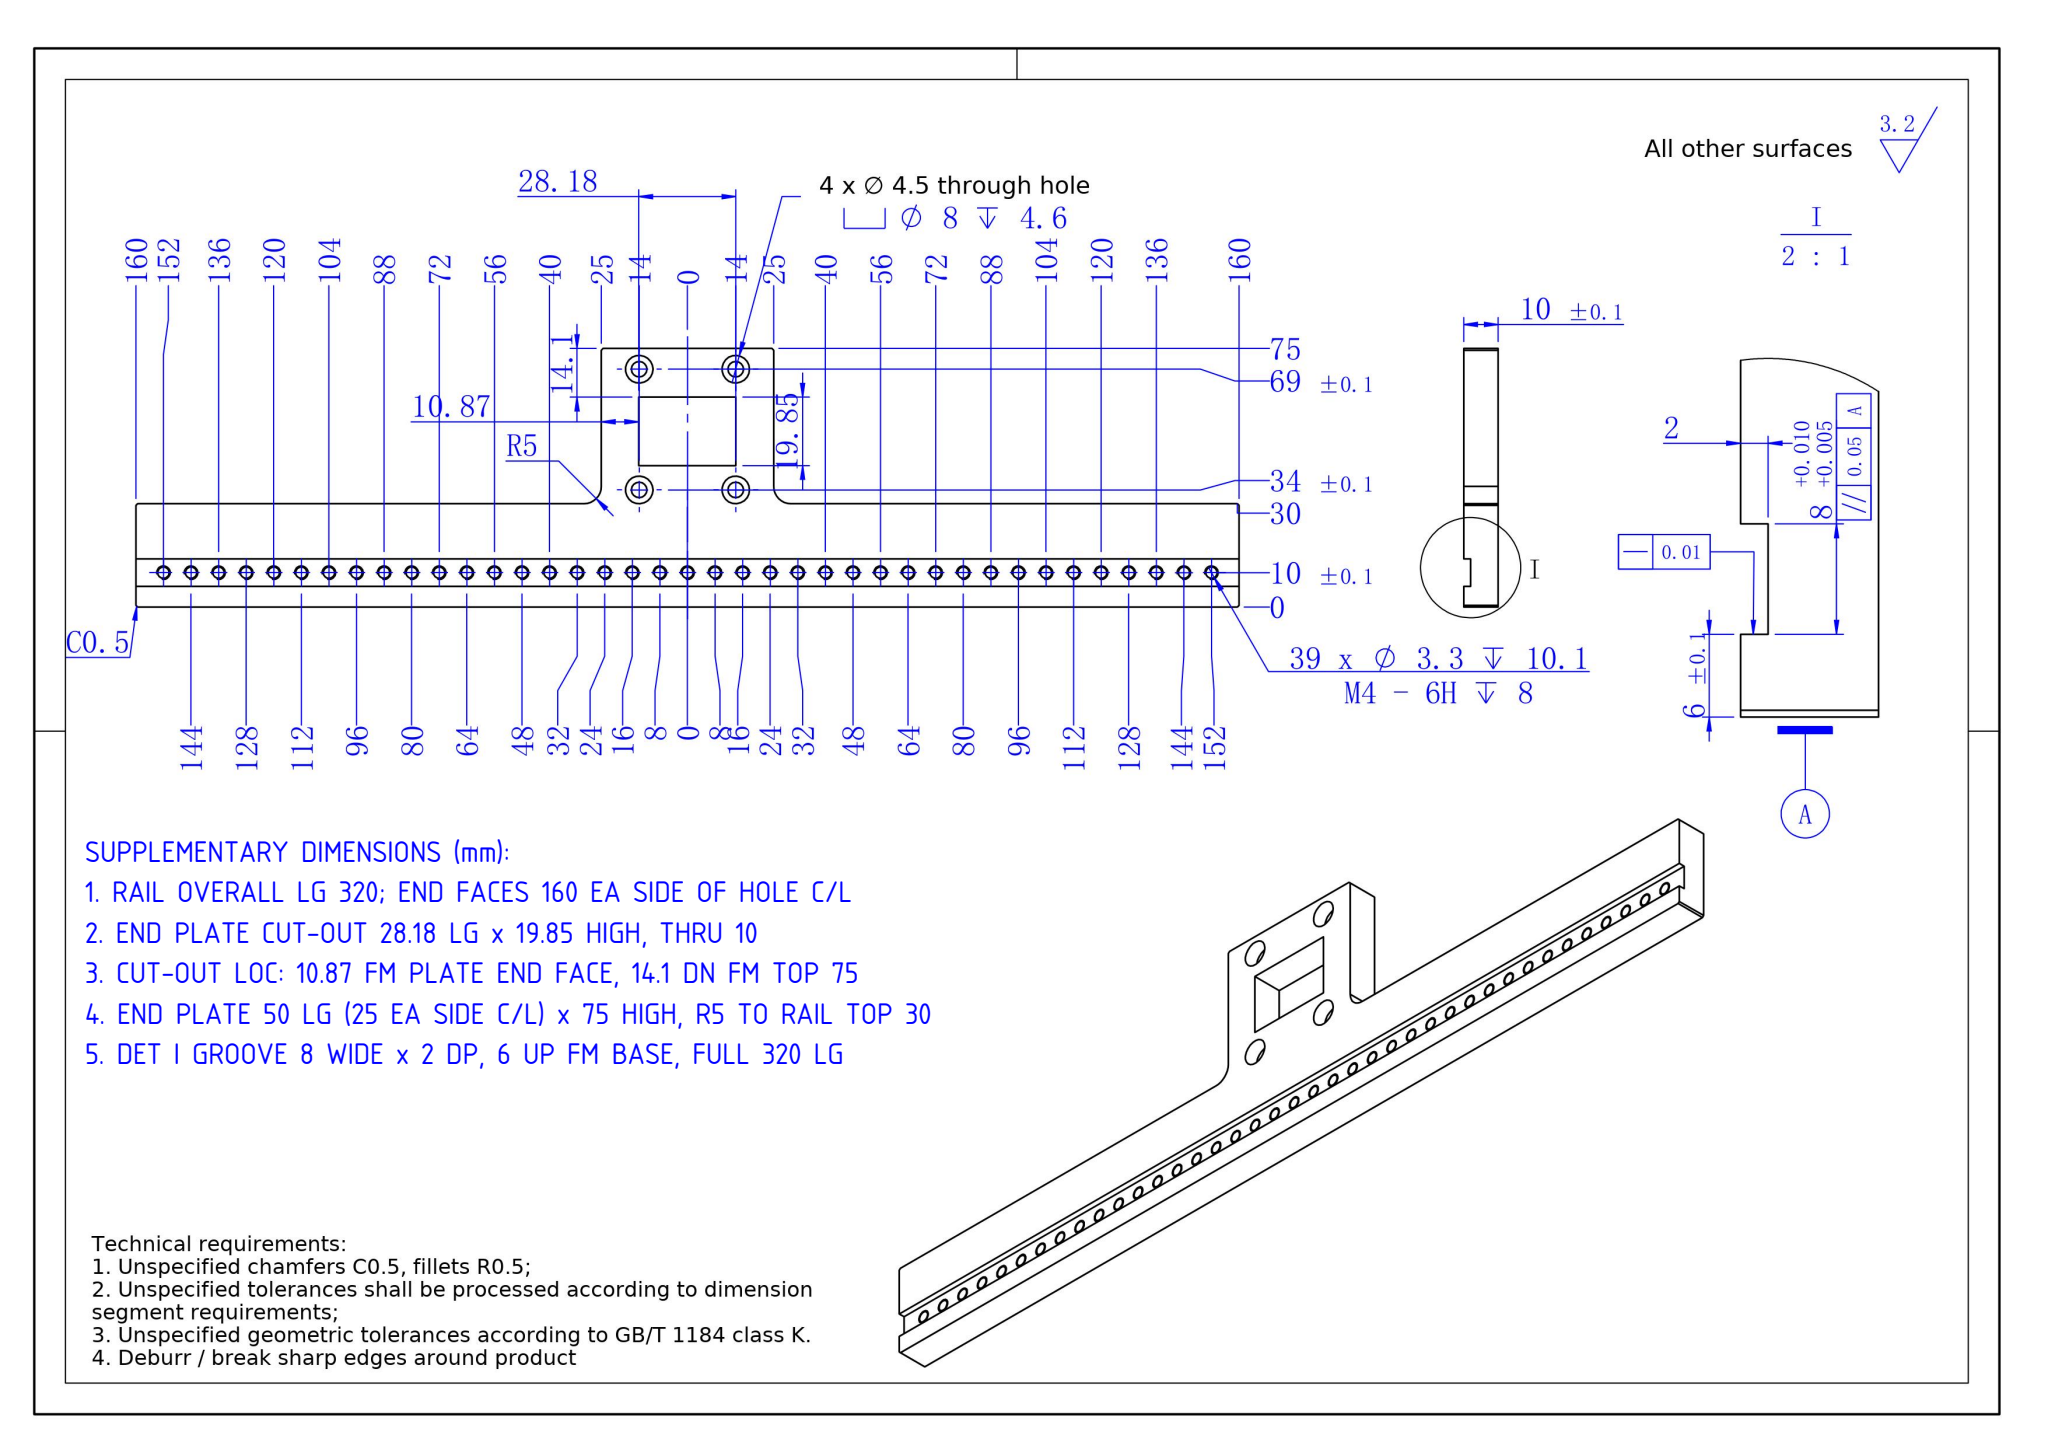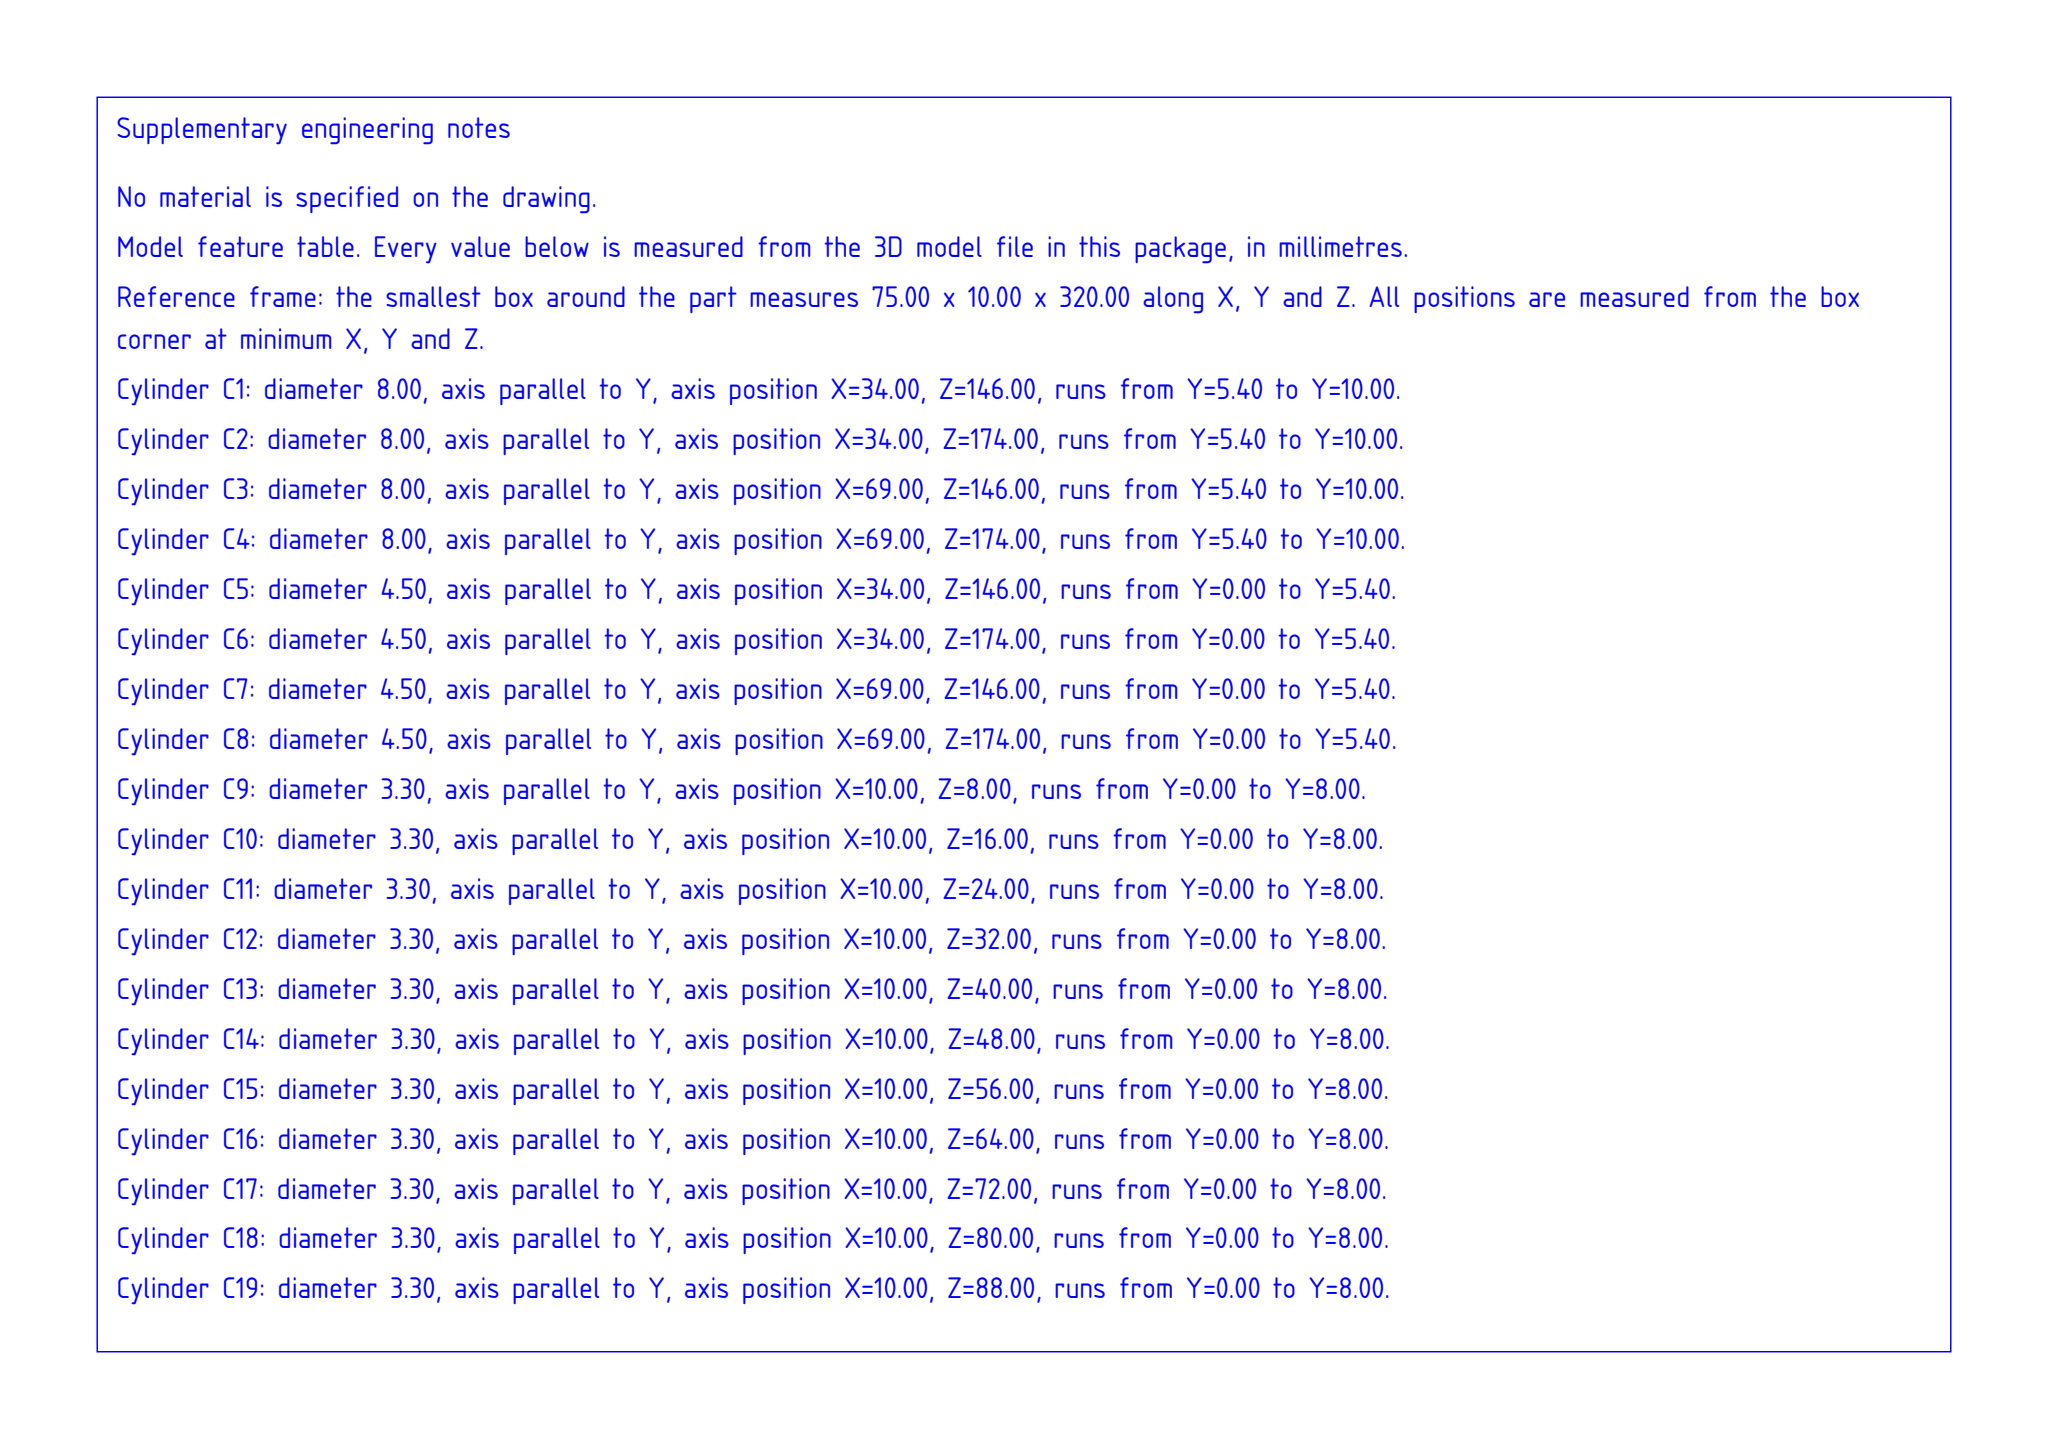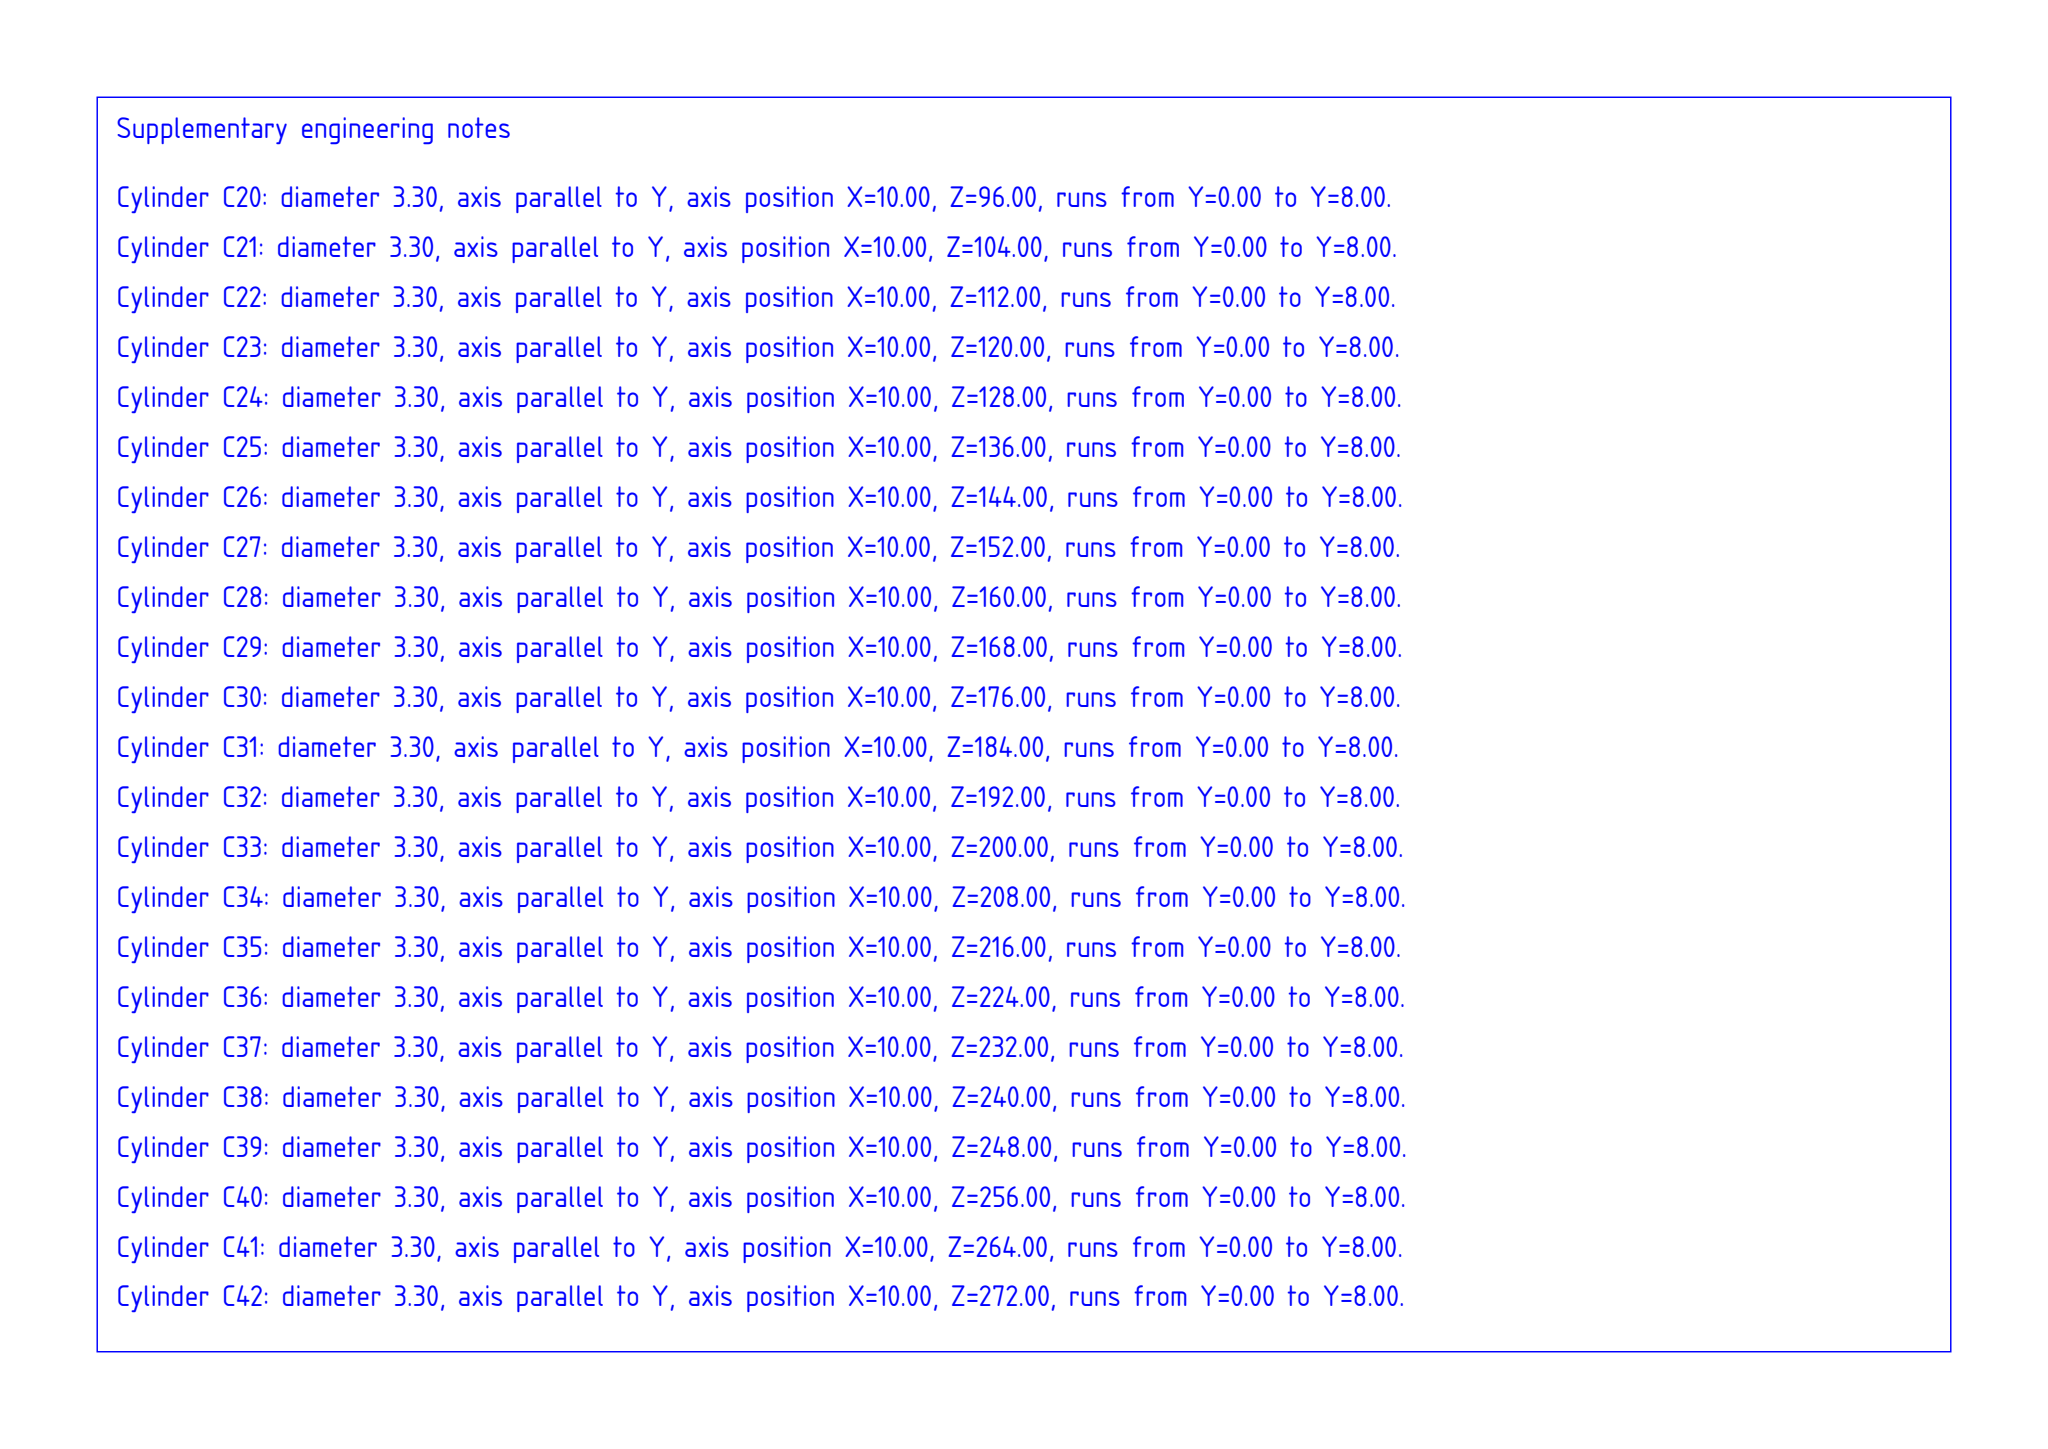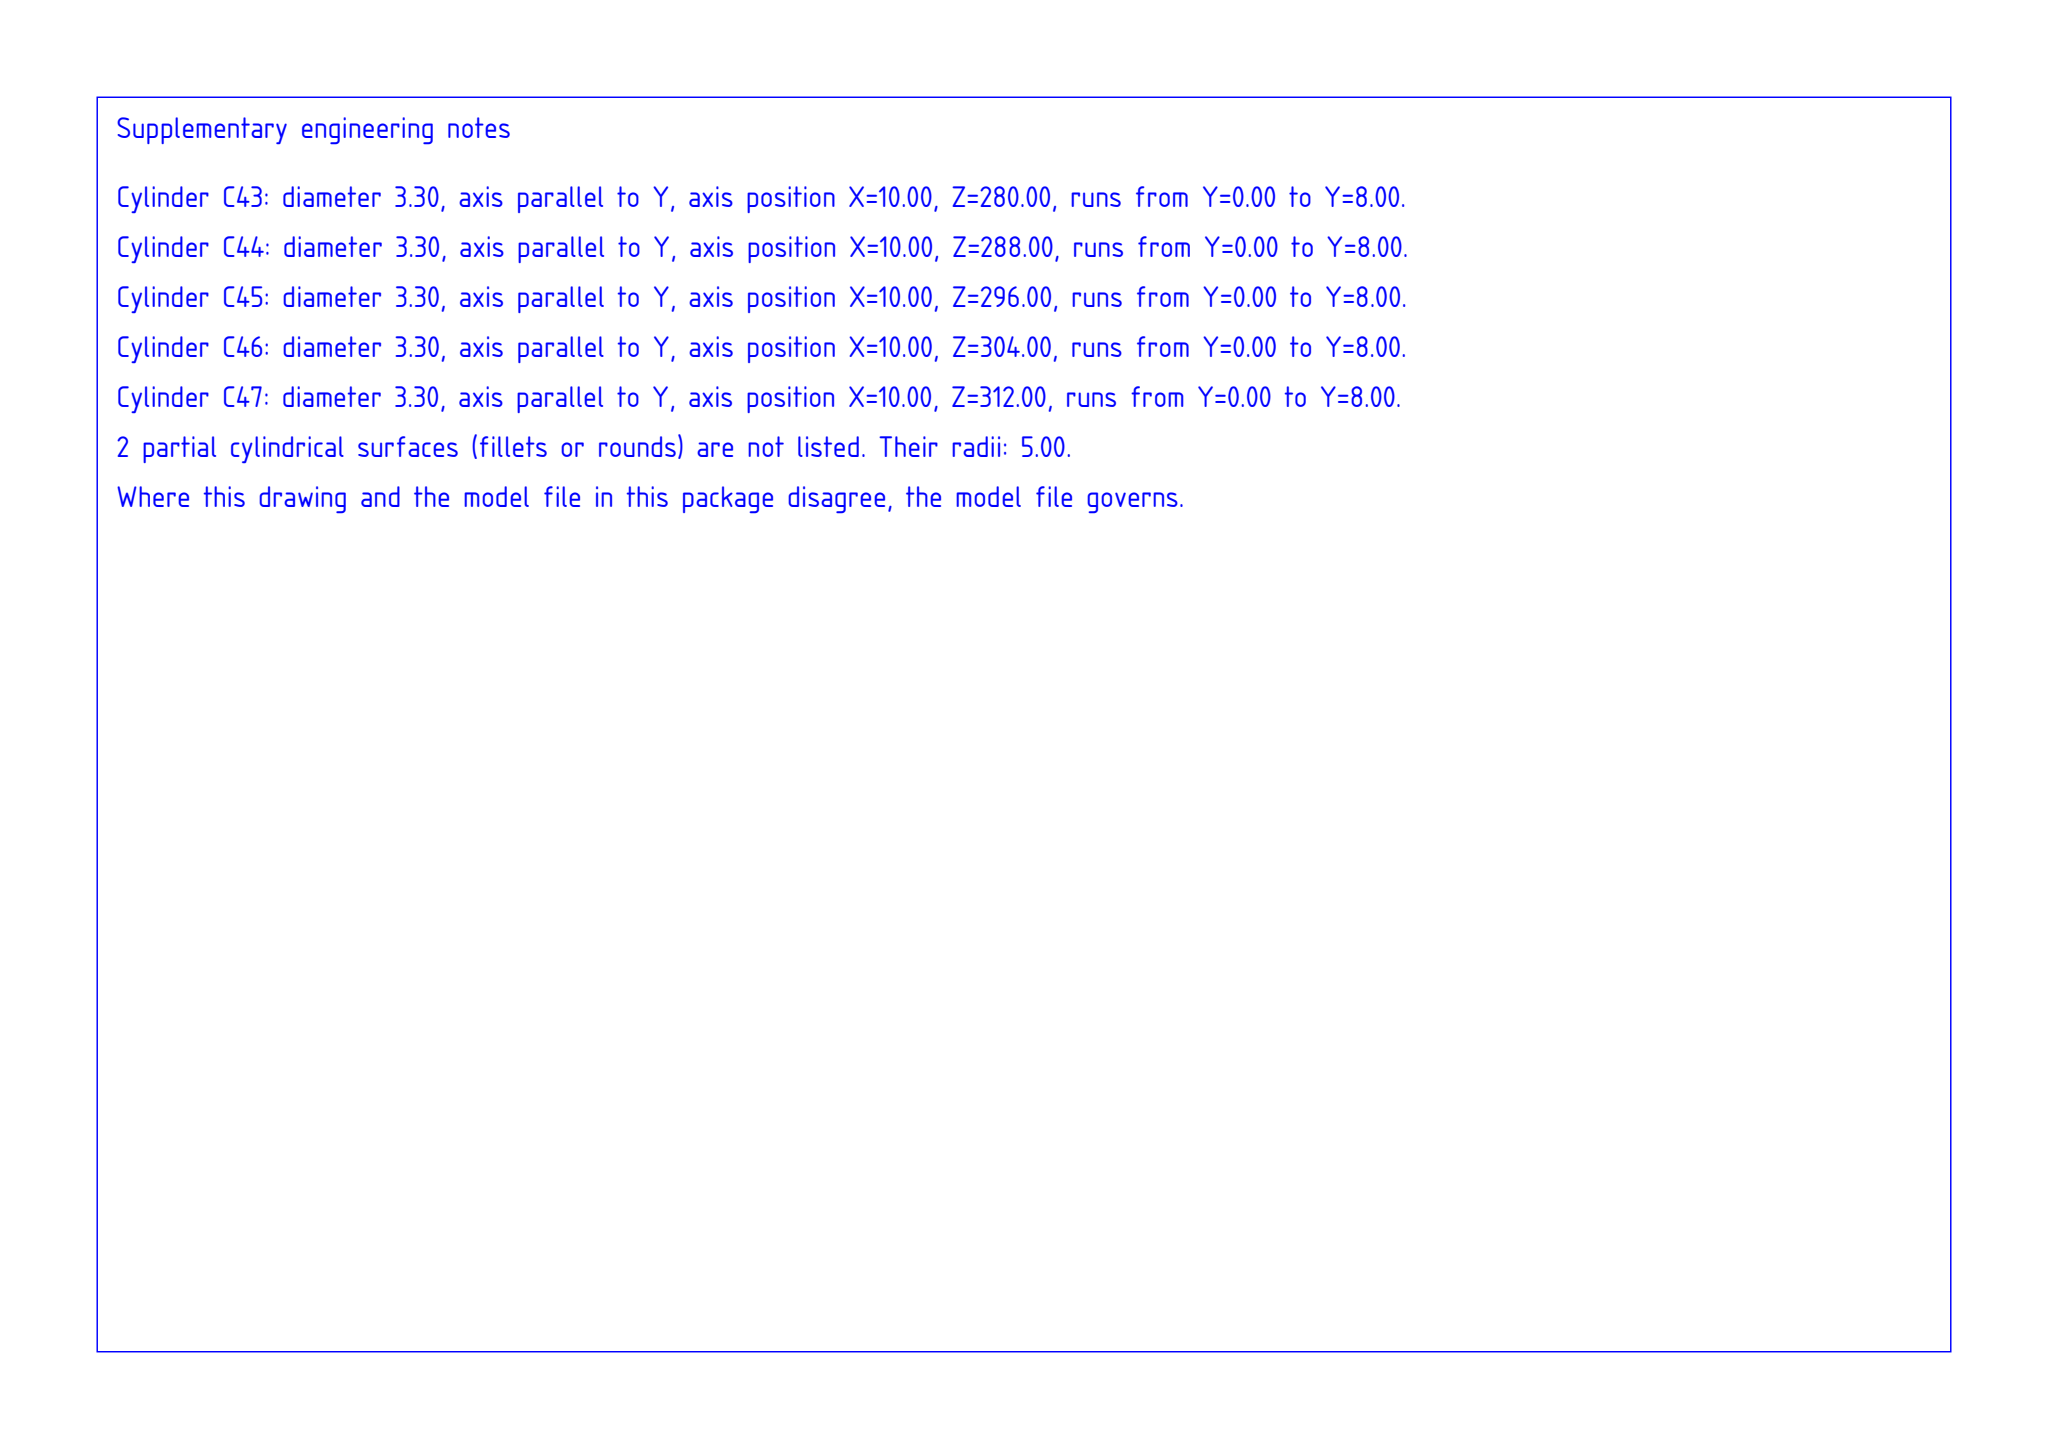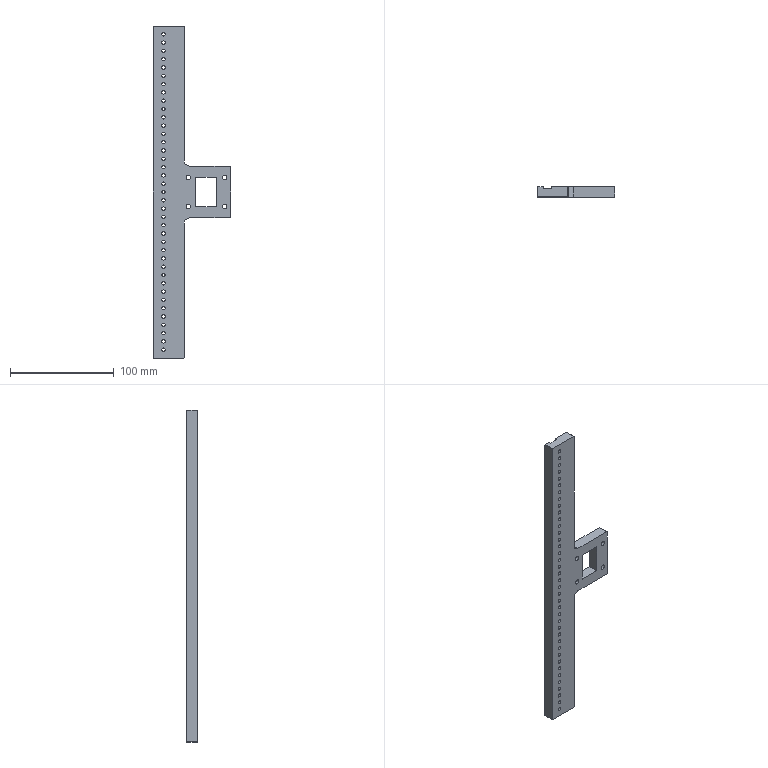Part | SolidWorks | mm | 1 solid | 124 faces | box 75 x 10 x 320 mm | volume 103950 mm3 | cylinder 96 | plane 28 | commonest cylinder face diameters 3.3 x78 8 x8 4.5 x8 10 x2
build123d program:
from build123d import *

# Parameters (mm, degrees)
SKETCH1_W                                          = 75
SKETCH1_H                                          = 10
BOSS_EXTRUDE1_DEPTH                                = 50
HOLE_SIZE_ACCORDING_TO_TYPE_1_OF_HEXAG_D           = 4.5
HOLE_SIZE_ACCORDING_TO_TYPE_1_OF_HEXAG_CBORE_D     = 8
HOLE_SIZE_ACCORDING_TO_TYPE_1_OF_HEXAG_CBORE_DEPTH = 4.6
SKETCH6_W                                          = 30
SKETCH6_H                                          = 135
BOSS_EXTRUDE2_DEPTH                                = 10
SKETCH8_W                                          = 8
SKETCH8_H                                          = 320
CUT_EXTRUDE1_DEPTH                                 = 2
FILLET1_R                                          = 5
LPATTERN2_COUNT                                    = 39
LPATTERN2_PITCH                                    = 8
CHAMFER1_SIZE                                      = 0.5
SKETCH11_W                                         = 19.847
SKETCH11_H                                         = 28.178
CUT_EXTRUDE2_DEPTH                                 = 60


with BuildPart() as part:
    # Sketch1 → Boss-Extrude1 (new body)
    with BuildSketch(Plane.XY):
        with Locations((-37.5, 5)):
            Rectangle(SKETCH1_W, SKETCH1_H)
    extrude(amount=BOSS_EXTRUDE1_DEPTH)

    # Hole Size _According to_ Type 1 of Hexag (through all)
    with Locations(Plane(origin=(-41, 10, 11), x_dir=(0, 0, 1), z_dir=(0, 1, 0))):
        with Locations((0, 0), (0, 35), (28, 35), (28, 0)):
            CounterBoreHole(HOLE_SIZE_ACCORDING_TO_TYPE_1_OF_HEXAG_D / 2, HOLE_SIZE_ACCORDING_TO_TYPE_1_OF_HEXAG_CBORE_D / 2, HOLE_SIZE_ACCORDING_TO_TYPE_1_OF_HEXAG_CBORE_DEPTH)

    # Sketch6 → Boss-Extrude2 (add)
    with BuildSketch(Plane(origin=(0, 10, 0), x_dir=(1, 0, 0), z_dir=(0, 1, 0))):
        with Locations((-60, 67.5)):
            Rectangle(SKETCH6_W, SKETCH6_H)
        with Locations((-60, -117.5)):
            Rectangle(SKETCH6_W, SKETCH6_H)
    extrude(amount=-BOSS_EXTRUDE2_DEPTH)

    # Sketch8 → Cut-Extrude1 (cut)
    with BuildSketch(Plane(origin=(0, 10, 0), x_dir=(1, 0, 0), z_dir=(0, 1, 0))):
        with Locations((-65, -25)):
            Rectangle(SKETCH8_W, SKETCH8_H)
    extrude(amount=-CUT_EXTRUDE1_DEPTH, mode=Mode.SUBTRACT)

    # Fillet1
    fillet1_edges = [part.edges().sort_by_distance(p)[0] for p in [
        (-45, 5, 0),
        (-45, 5, 50),
    ]]
    fillet(fillet1_edges, radius=FILLET1_R)

    # Sketch10 → M4 Tapped Hole1 (revolve, cut)
    with BuildSketch(Plane(origin=(-65, 8, 177), x_dir=(0, 0, 1), z_dir=(1, 0, 0))):
        Polygon((0, 0), (0, 11.091), (1.65, 10.1), (1.65, 0), align=None)
    m4_tapped_hole1 = revolve(axis=Axis((-65, 14.35, 177), (0, -1, 0)), mode=Mode.SUBTRACT)

    # LPattern2: M4 Tapped Hole1 ×39
    with Locations(*[(0, 0, -i * LPATTERN2_PITCH) for i in range(1, LPATTERN2_COUNT)]):
        add(m4_tapped_hole1, mode=Mode.SUBTRACT)

    # Chamfer1
    chamfer1_edges = [part.edges().sort_by_distance(p)[0] for p in [
        (0, 5, 50),
        (0, 5, 0),
        (-45, 5, -135),
        (-75, 5, -135),
        (-45, 5, 185),
        (-75, 5, 185),
    ]]
    chamfer(chamfer1_edges, length=CHAMFER1_SIZE)

    # Sketch11 → Cut-Extrude2 (cut)
    with BuildSketch(Plane(origin=(0, 10, 0), x_dir=(1, 0, 0), z_dir=(0, 1, 0))):
        with Locations((-24.022, -24.962)):
            Rectangle(SKETCH11_W, SKETCH11_H)
    extrude(amount=-CUT_EXTRUDE2_DEPTH, mode=Mode.SUBTRACT)


solid = part.part